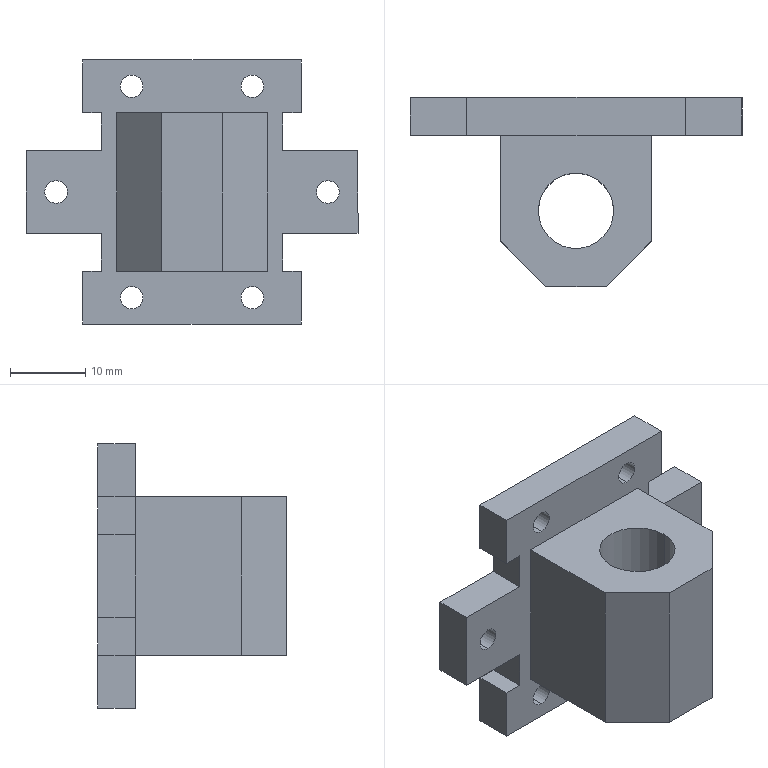Component | SolidWorks | 618-8BearingHousing-1 | 1 solid | 43 faces | box 44 x 25 x 35 mm | volume 11433 mm3 | plane 29 | cylinder 14 | commonest cylinder face diameters 3 x12 10 x2 | material 6061 Alloy
build123d program:
from build123d import *

# Parameters (mm, degrees)
SKETCH3_R           = 5
BOSS_EXTRUDE1_DEPTH = 17.5
SKETCH5_W           = 9
SKETCH5_H           = 5
SKETCH5_R           = 1.5
CUT_EXTRUDE2_DEPTH  = 34.871
SKETCH8_W           = 6.5
SKETCH8_H           = 7
CUT_EXTRUDE5_DEPTH  = 38.044
SKETCH9_W           = 20
SKETCH9_H           = 20
CUT_EXTRUDE6_DEPTH  = 7
CHAMFER1_SIZE       = 6
SKETCH10_W          = 11
SKETCH10_H          = 5
BOSS_EXTRUDE2_DEPTH = 1
SKETCH11_W          = 11
SKETCH11_H          = 5
BOSS_EXTRUDE3_DEPTH = 1


with BuildPart() as part:
    # Sketch3 → Boss-Extrude1 (new, symmetric)
    with BuildSketch(Plane.XY):
        Polygon((-10, 12.5), (-10, 2.5), (-21, 2.5), (-21, -2.5), (21, -2.5), (21, 2.5), (10, 2.5), (10, 12.5), (10, 22.5), (-10, 22.5), align=None)
        with Locations((0, 12.5)):
            Circle(SKETCH3_R, mode=Mode.SUBTRACT)
    extrude(amount=BOSS_EXTRUDE1_DEPTH, both=True)

    # Sketch5 → Cut-Extrude2 (cut, through all)
    with BuildSketch(Plane(origin=(0, 2.5, 0), x_dir=(1, 0, 0), z_dir=(0, 1, 0))):
        with Locations((-16.5, 8)):
            Rectangle(SKETCH5_W, SKETCH5_H)
        with Locations((16.5, 8)):
            Rectangle(SKETCH5_W, SKETCH5_H)
        with Locations((16.5, -8)):
            Rectangle(SKETCH5_W, SKETCH5_H)
        with Locations((-16.5, -8)):
            Rectangle(SKETCH5_W, SKETCH5_H)
        with Locations(Location((-8, 14, 0), (0, 0, 270))):
            Circle(SKETCH5_R)
        with Locations(Location((8, 14, 0), (0, 0, 270))):
            Circle(SKETCH5_R)
        with Locations(Location((-8, -14, 0), (0, 0, 270))):
            Circle(SKETCH5_R)
        with Locations(Location((8, -14, 0), (0, 0, 270))):
            Circle(SKETCH5_R)
        with Locations(Location((18, 0, 0), (0, 0, 270))):
            Circle(SKETCH5_R)
        with Locations(Location((-18, 0, 0), (0, 0, 270))):
            Circle(SKETCH5_R)
    extrude(amount=-CUT_EXTRUDE2_DEPTH, mode=Mode.SUBTRACT)

    # Sketch8 → Cut-Extrude5 (cut, through all)
    with BuildSketch(Plane.XZ.offset(2.5)):
        with Locations((-17.75, 14)):
            Rectangle(SKETCH8_W, SKETCH8_H)
        with Locations((-17.75, -14)):
            Rectangle(SKETCH8_W, SKETCH8_H)
        with Locations((17.75, -14)):
            Rectangle(SKETCH8_W, SKETCH8_H)
        with Locations((17.75, 14)):
            Rectangle(SKETCH8_W, SKETCH8_H)
    extrude(amount=-CUT_EXTRUDE5_DEPTH, mode=Mode.SUBTRACT)

    # Sketch9 → Cut-Extrude6 (cut)
    with BuildSketch(Plane.XY.offset(17.5)):
        with Locations((0, 12.5)):
            Rectangle(SKETCH9_W, SKETCH9_H)
    cut_extrude6 = extrude(amount=-CUT_EXTRUDE6_DEPTH, mode=Mode.SUBTRACT)

    # Mirror1: Cut-Extrude6 across plane
    add(cut_extrude6.mirror(Plane.XY), mode=Mode.SUBTRACT)

    # Chamfer1
    chamfer1_edges = [part.edges().sort_by_distance(p)[0] for p in [
        (-10, 22.5, 0),
        (10, 22.5, 0),
    ]]
    chamfer(chamfer1_edges, length=CHAMFER1_SIZE)

    # Sketch10 → Boss-Extrude2 (add)
    with BuildSketch(Plane.ZY.offset(21)):
        Rectangle(SKETCH10_W, SKETCH10_H)
    extrude(amount=BOSS_EXTRUDE2_DEPTH)

    # Sketch11 → Boss-Extrude3 (add)
    with BuildSketch(Plane(origin=(21, 0, 0), x_dir=(0, 0, -1), z_dir=(1, 0, 0))):
        Rectangle(SKETCH11_W, SKETCH11_H)
    extrude(amount=BOSS_EXTRUDE3_DEPTH)


solid = part.part

# Placed as in the assembly
solid = solid.moved(Location((1.903, -15.483, 42), (180, 0, 0)))